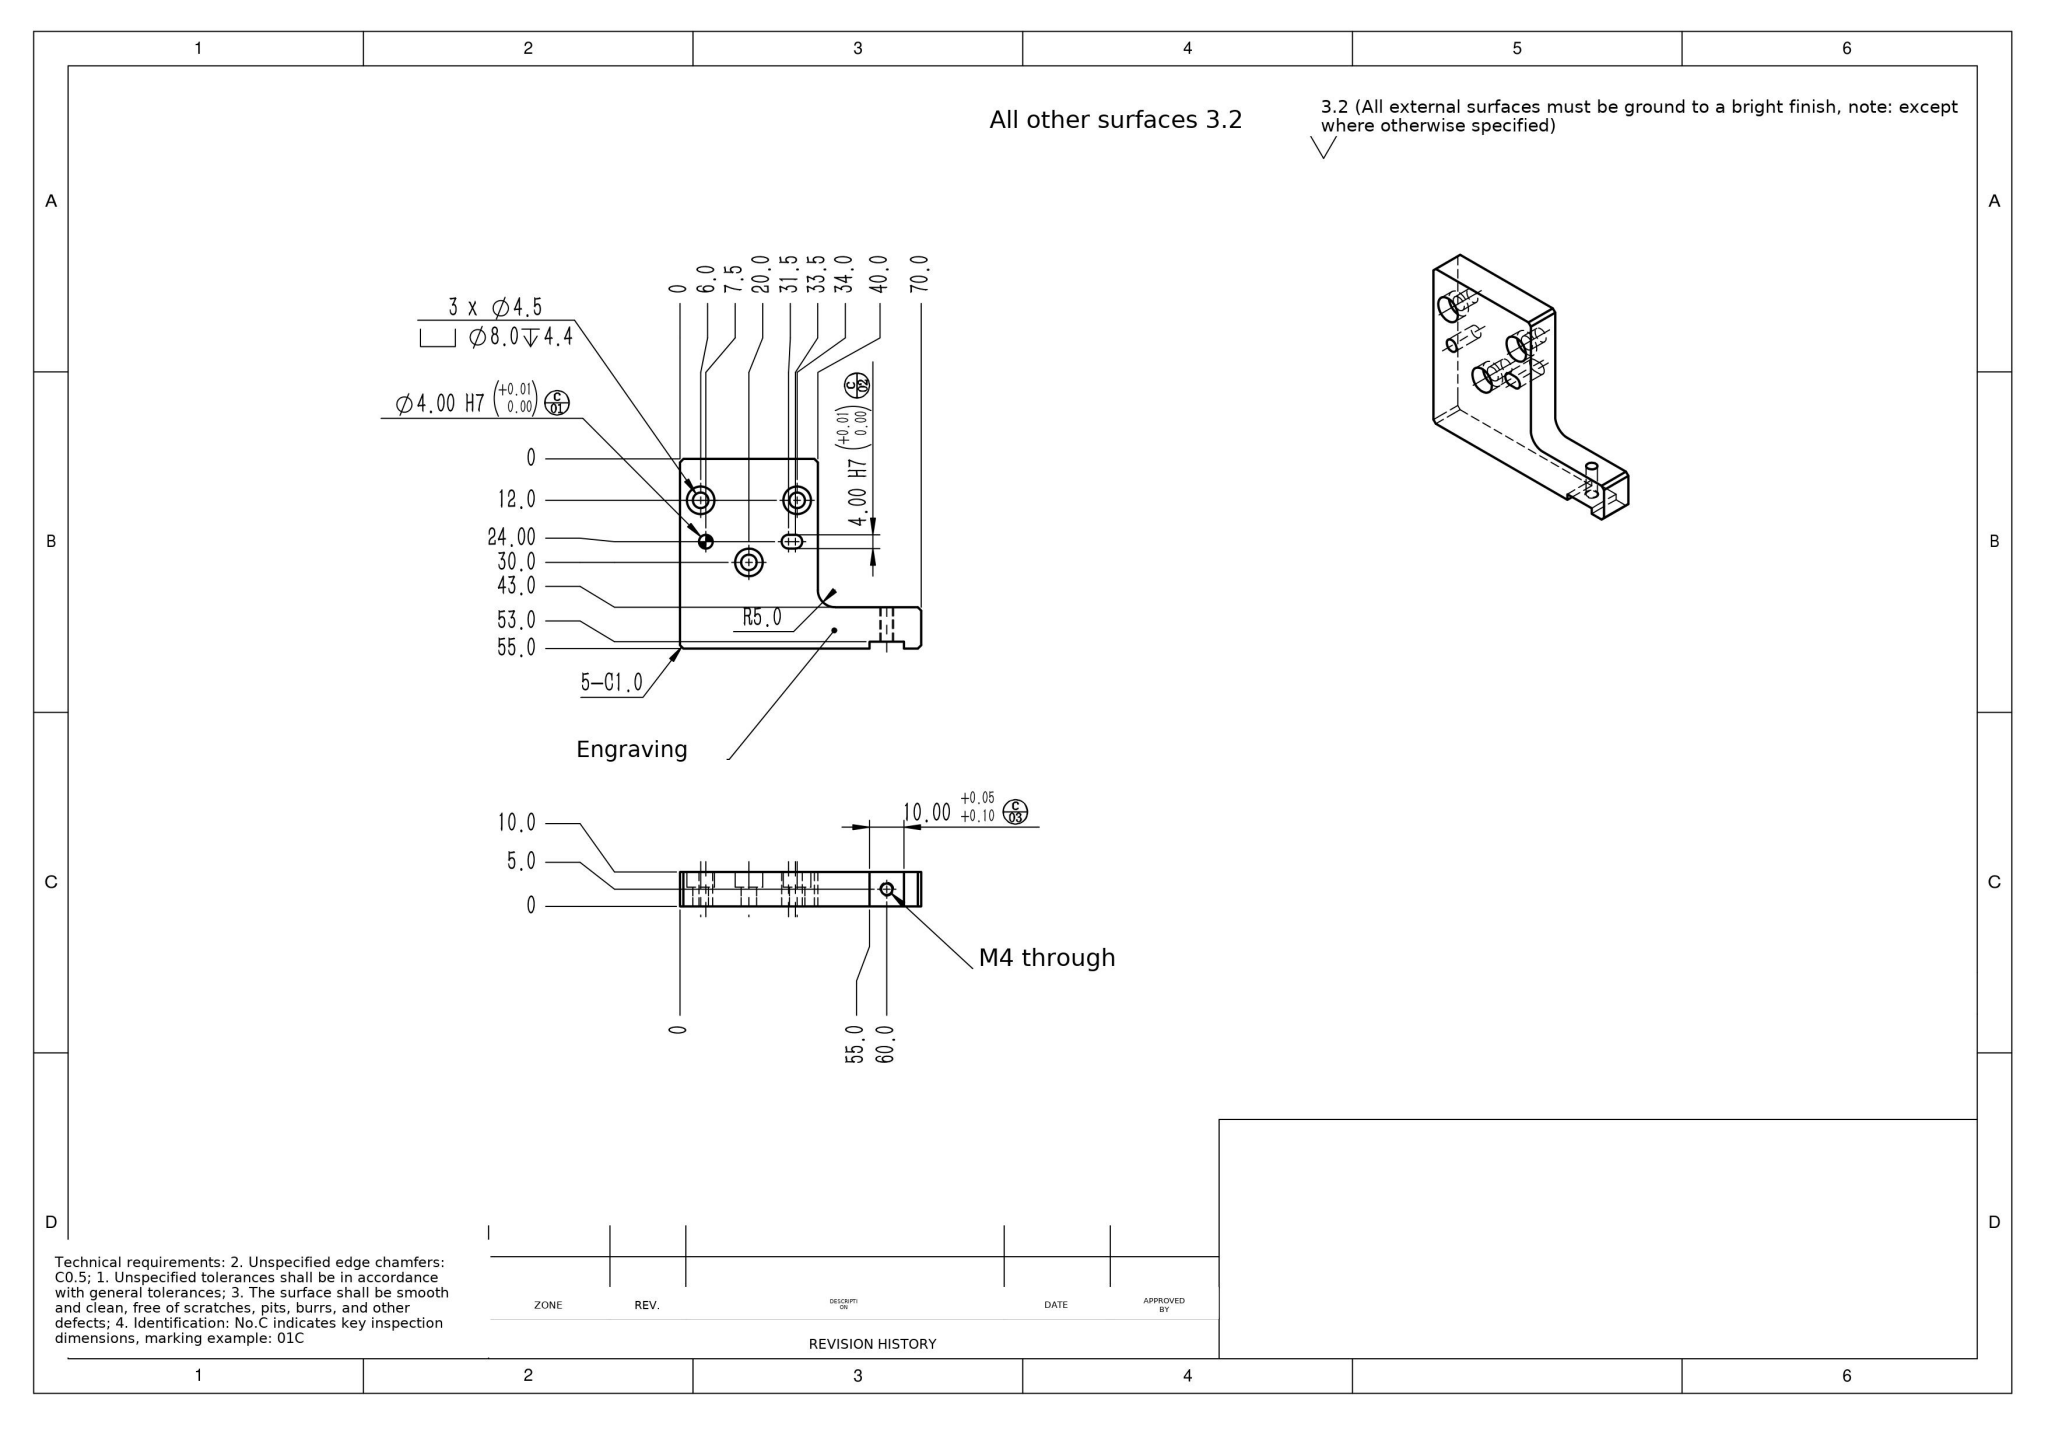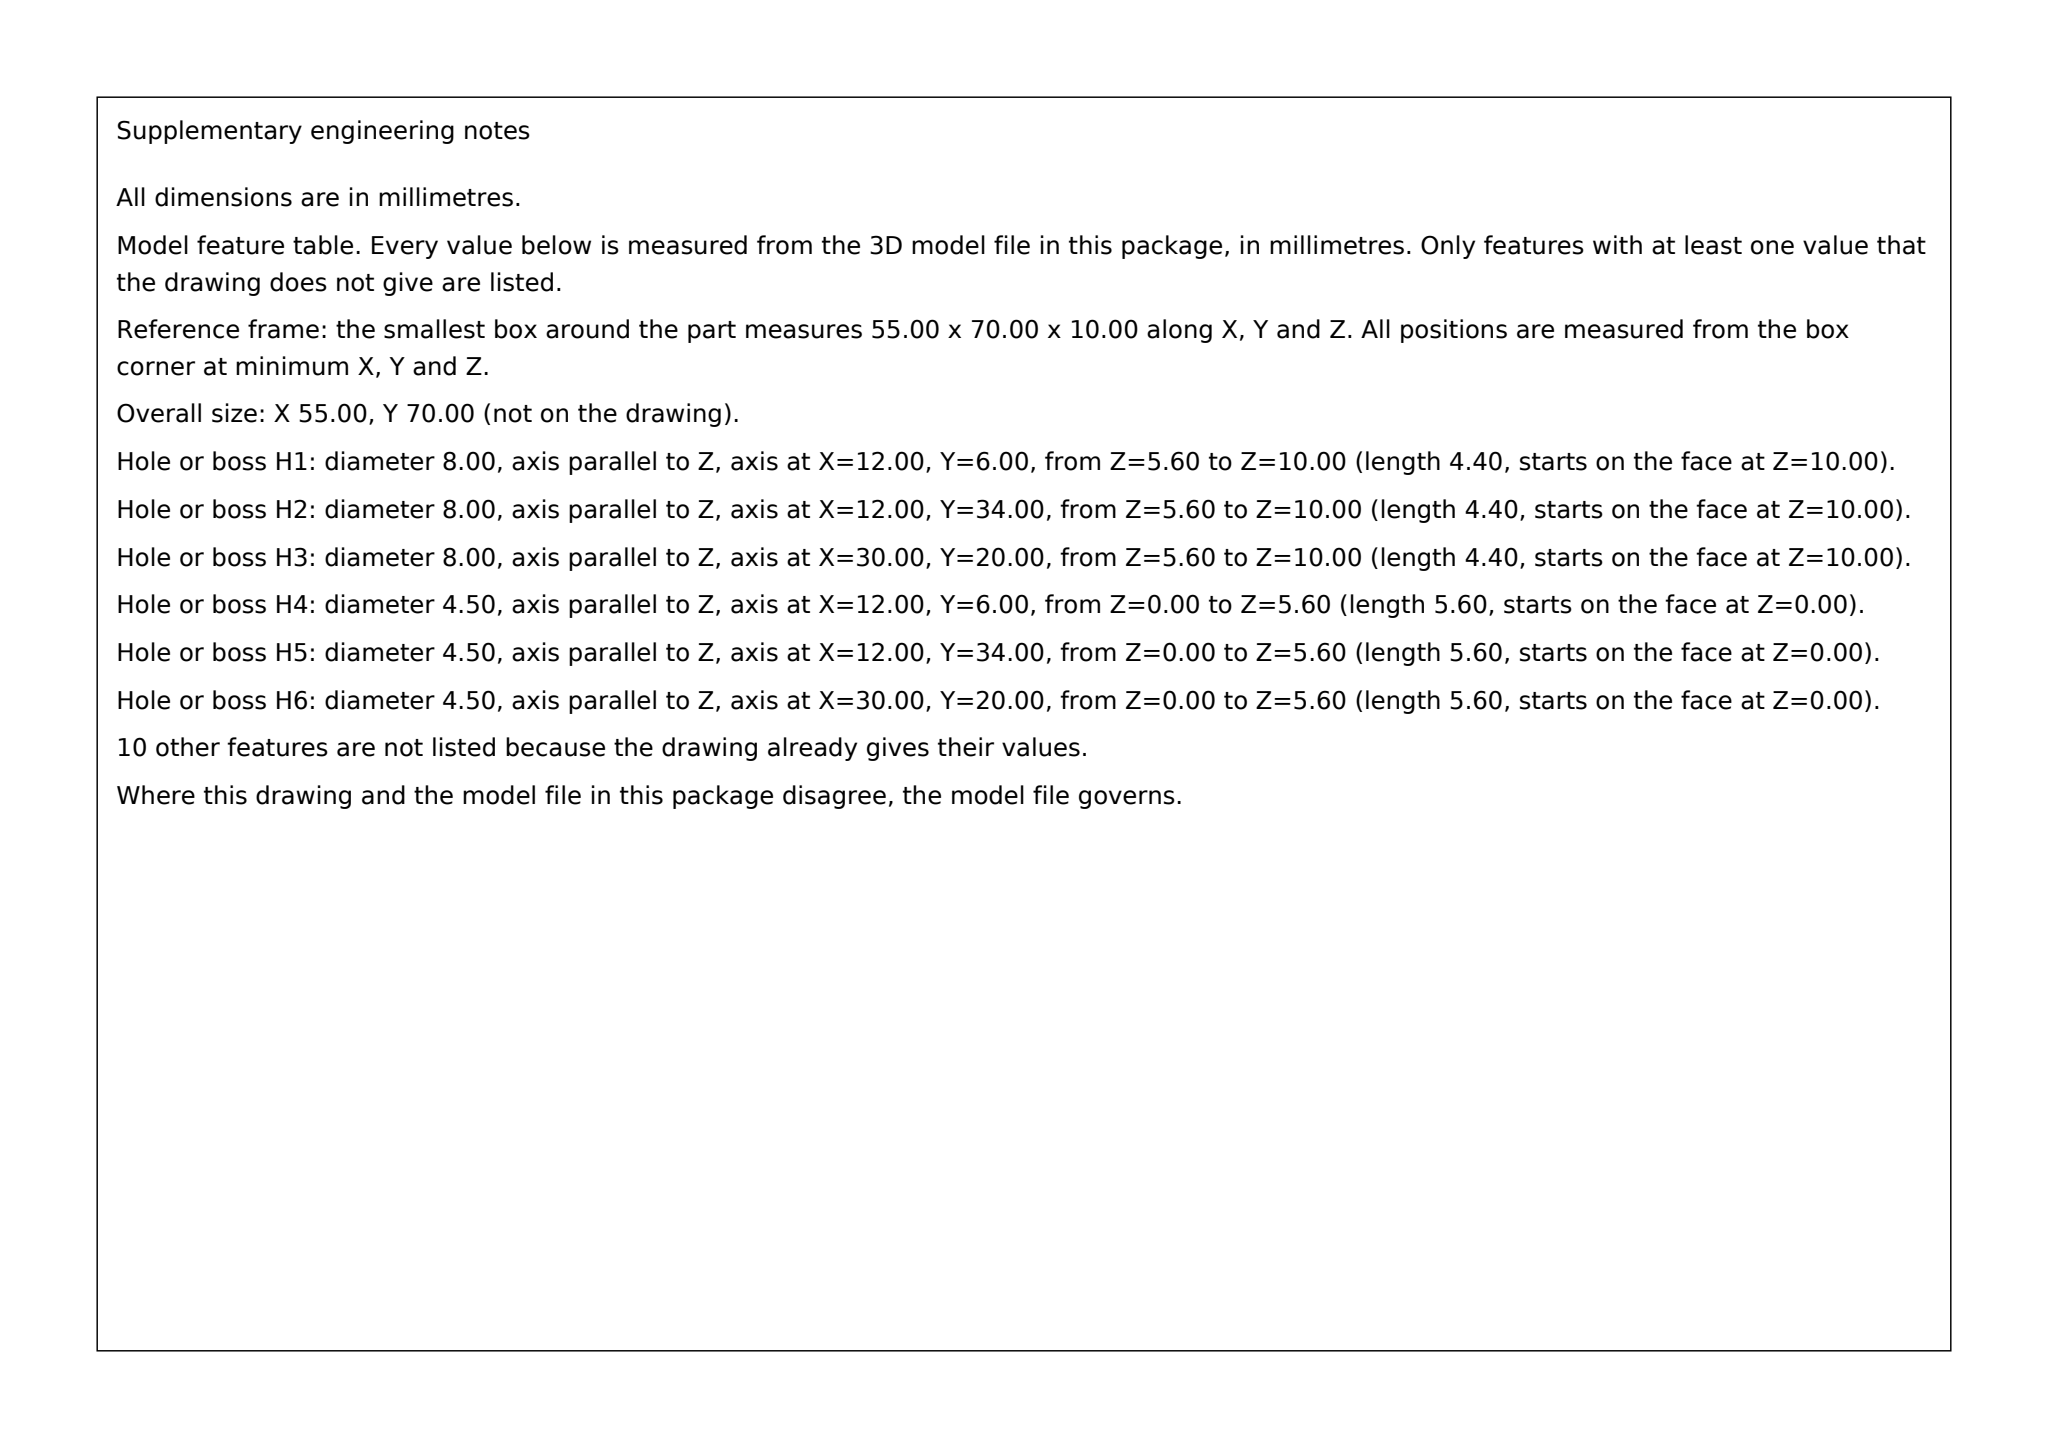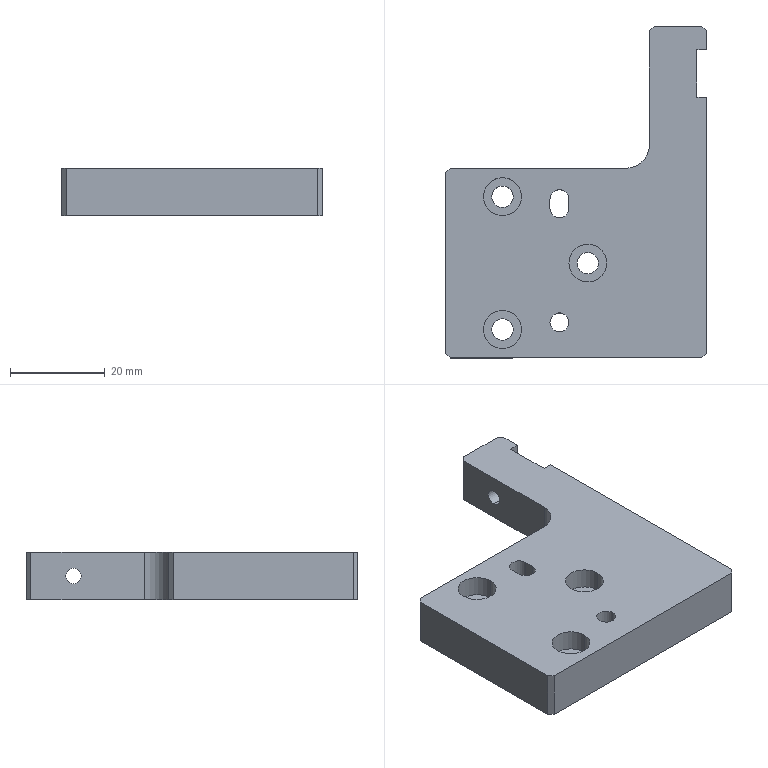Part | SolidWorks | mm | 1 solid | 41 faces | box 55 x 70 x 10 mm | volume 24081 mm3 | plane 22 | cylinder 19 | commonest cylinder face diameters 8 x6 4.5 x6 4 x4 3.3 x2 10 x1
build123d program:
from build123d import *

# Parameters (mm, degrees)
SKETCH1_W                                       = 55
SKETCH1_H                                       = 150
BOSS_EXTRUDE1_DEPTH                             = 10
SKETCH2_W                                       = 43
SKETCH2_H                                       = 110
CUT_EXTRUDE1_DEPTH                              = 10
SKETCH3_W                                       = 10
SKETCH3_H                                       = 80
CUT_EXTRUDE2_DEPTH                              = 94.541
FILLET1_R                                       = 5
CHAMFER2_SIZE                                   = 1
SKETCH5_W                                       = 10
SKETCH5_H                                       = 10
CUT_EXTRUDE6_DEPTH                              = 2
M4_TAPPED_HOLE1_D                               = 3.3
M4_HEX_SOCKET_HEAD_CAP_SCREW_CBORE1_D           = 4.5
M4_HEX_SOCKET_HEAD_CAP_SCREW_CBORE1_CBORE_D     = 8
M4_HEX_SOCKET_HEAD_CAP_SCREW_CBORE1_CBORE_DEPTH = 4.4
SKETCH10_R                                      = 2
CUT_EXTRUDE7_DEPTH                              = 81.506
CHAMFER3_SIZE                                   = 1


with BuildPart() as part:
    # Sketch1 → Boss-Extrude1 (new body)
    with BuildSketch(Plane.XY):
        Rectangle(SKETCH1_W, SKETCH1_H)
    extrude(amount=BOSS_EXTRUDE1_DEPTH)

    # Sketch2 → Cut-Extrude1 (cut)
    with BuildSketch(Plane.XY.offset(10)):
        with Locations((-6, 20)):
            Rectangle(SKETCH2_W, SKETCH2_H)
    extrude(amount=-CUT_EXTRUDE1_DEPTH, mode=Mode.SUBTRACT)

    # Sketch3 → Cut-Extrude2 (cut, through all)
    with BuildSketch(Plane(origin=(27.5, 0, 0), x_dir=(0, 0, -1), z_dir=(1, 0, 0))):
        with Locations((-5, 35)):
            Rectangle(SKETCH3_W, SKETCH3_H)
    extrude(amount=-CUT_EXTRUDE2_DEPTH, mode=Mode.SUBTRACT)

    # Fillet1
    fillet1_edges = [part.edges().sort_by_distance(p)[0] for p in [
        (15.5, -35, 5),
    ]]
    fillet(fillet1_edges, radius=FILLET1_R)

    # Chamfer2
    chamfer2_edges = [part.edges().sort_by_distance(p)[0] for p in [
        (-27.5, -35, 5),
        (27.5, -75, 5),
        (-27.5, -75, 5),
    ]]
    chamfer(chamfer2_edges, length=CHAMFER2_SIZE)

    # Sketch5 → Cut-Extrude6 (cut)
    with BuildSketch(Plane(origin=(27.5, 0, 0), x_dir=(0, 0, -1), z_dir=(1, 0, 0))):
        with Locations((-5, -15)):
            Rectangle(SKETCH5_W, SKETCH5_H)
    extrude(amount=-CUT_EXTRUDE6_DEPTH, mode=Mode.SUBTRACT)

    # M4 Tapped Hole1 (through all)
    with Locations(Plane(origin=(25.5, 0, 0), x_dir=(0, 0, -1), z_dir=(1, 0, 0))):
        with Locations((-5, -15)):
            Hole(M4_TAPPED_HOLE1_D / 2)

    # M4 Hex Socket Head Cap Screw CBORE1 (through all)
    with Locations(Plane.XY.offset(10)):
        with Locations((-15.5, -41), (-15.5, -69), (2.5, -55)):
            CounterBoreHole(M4_HEX_SOCKET_HEAD_CAP_SCREW_CBORE1_D / 2, M4_HEX_SOCKET_HEAD_CAP_SCREW_CBORE1_CBORE_D / 2, M4_HEX_SOCKET_HEAD_CAP_SCREW_CBORE1_CBORE_DEPTH)

    # Sketch10 → Cut-Extrude7 (cut, through all)
    with BuildSketch(Plane.XY.offset(10)):
        with Locations((-3.5, -67.5)):
            Circle(SKETCH10_R)
        with BuildLine():
            Line((-5.5, -43.5), (-5.5, -41.5))
            ThreePointArc((-5.5, -41.5), (-3.5, -39.5), (-1.5, -41.5))
            Line((-1.5, -41.5), (-1.5, -43.5))
            ThreePointArc((-1.5, -43.5), (-3.5, -45.5), (-5.5, -43.5))
        make_face()
    extrude(amount=-CUT_EXTRUDE7_DEPTH, mode=Mode.SUBTRACT)

    # Chamfer3
    chamfer3_edges = [part.edges().sort_by_distance(p)[0] for p in [
        (15.5, -5, 5),
        (27.5, -5, 5),
    ]]
    chamfer(chamfer3_edges, length=CHAMFER3_SIZE)


solid = part.part